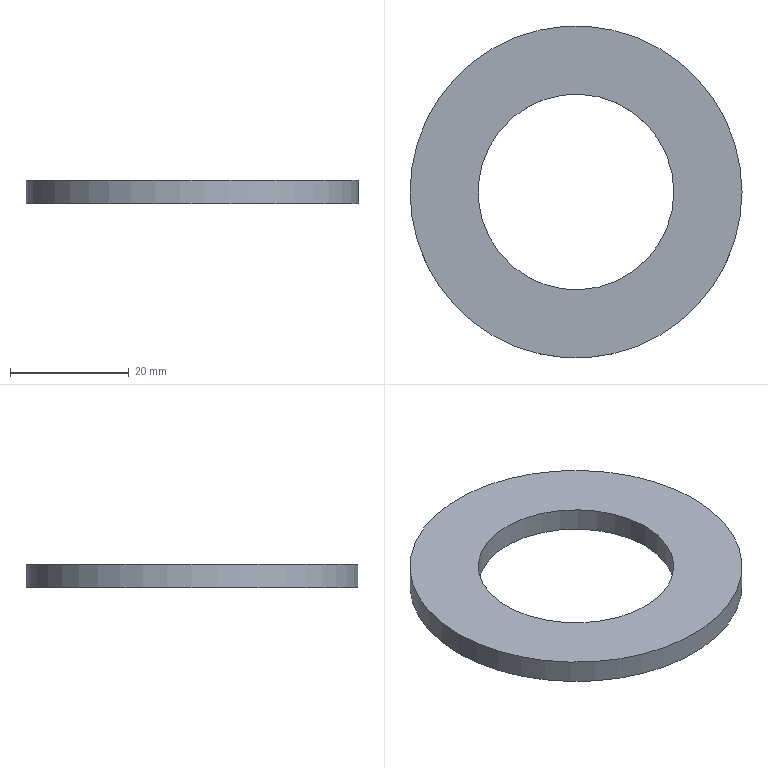Component | NX | GB-T95-2002_M30 | 1 solid | 4 faces | box 56 x 56 x 4 mm | volume 6431 mm3 | cylinder 2 | plane 2 | commonest cylinder face diameters 56 x1 33 x1
STEP:
#1=CARTESIAN_POINT('',(0.,0.,0.));
#2=DIRECTION('',(0.,0.,1.));
#3=DIRECTION('',(1.,0.,0.));
#4=AXIS2_PLACEMENT_3D('',#1,#2,#3);
#5=CARTESIAN_POINT('',(28.,0.,-9.));
#6=VERTEX_POINT('',#5);
#7=CARTESIAN_POINT('',(0.,0.,-9.));
#8=DIRECTION('',(0.,0.,1.));
#9=DIRECTION('',(1.,0.,0.));
#10=AXIS2_PLACEMENT_3D('',#7,#8,#9);
#11=CIRCLE('',#10,28.);
#12=CARTESIAN_POINT('',(0.,0.,-5.));
#13=DIRECTION('',(0.,0.,1.));
#14=DIRECTION('',(1.,0.,0.));
#15=AXIS2_PLACEMENT_3D('',#12,#13,#14);
#16=CYLINDRICAL_SURFACE('',#15,28.);
#17=CARTESIAN_POINT('',(0.,-4.));
#18=DIRECTION('',(1.,0.));
#19=VECTOR('',#18,1.);
#20=LINE('',#17,#19);
#21=(GEOMETRIC_REPRESENTATION_CONTEXT(2)PARAMETRIC_REPRESENTATION_CONTEXT()REPRESENTATION_CONTEXT('',''));
#22=DEFINITIONAL_REPRESENTATION('',(#20),#21);
#23=PCURVE('',#16,#22);
#24=CARTESIAN_POINT('',(-28.,0.,-9.));
#25=DIRECTION('',(0.,0.,-1.));
#26=DIRECTION('',(-1.,0.,0.));
#27=AXIS2_PLACEMENT_3D('',#24,#25,#26);
#28=PLANE('',#27);
#29=CARTESIAN_POINT('',(-56.,0.));
#30=CARTESIAN_POINT('',(-56.,48.497));
#31=CARTESIAN_POINT('',(-14.,24.249));
#32=CARTESIAN_POINT('',(28.,0.));
#33=CARTESIAN_POINT('',(-14.,-24.249));
#34=CARTESIAN_POINT('',(-56.,-48.497));
#35=CARTESIAN_POINT('',(-56.,0.));
#36=(BOUNDED_CURVE()B_SPLINE_CURVE(2,(#29,#30,#31,#32,#33,#34,#35),.UNSPECIFIED.,.T.,.F.)B_SPLINE_CURVE_WITH_KNOTS((1,2,2,2,2,1),(-2.094,0.,2.094,4.189,6.283,8.378),.UNSPECIFIED.)CURVE()GEOMETRIC_REPRESENTATION_ITEM()RATIONAL_B_SPLINE_CURVE((1.,0.5,1.,0.5,1.,0.5,1.))REPRESENTATION_ITEM(''));
#37=(GEOMETRIC_REPRESENTATION_CONTEXT(2)PARAMETRIC_REPRESENTATION_CONTEXT()REPRESENTATION_CONTEXT('',''));
#38=DEFINITIONAL_REPRESENTATION('',(#36),#37);
#39=PCURVE('',#28,#38);
#40=SURFACE_CURVE('',#11,(#23,#39),.PCURVE_S1.);
#41=EDGE_CURVE('',#6,#6,#40,.T.);
#42=ORIENTED_EDGE('',*,*,#41,.T.);
#43=CARTESIAN_POINT('',(28.,0.,-5.));
#44=VERTEX_POINT('',#43);
#45=CARTESIAN_POINT('',(28.,0.,-9.));
#46=CARTESIAN_POINT('',(28.,0.,-5.));
#47=B_SPLINE_CURVE_WITH_KNOTS('',1,(#45,#46),.UNSPECIFIED.,.F.,.F.,(2,2),(-4.,0.),.PIECEWISE_BEZIER_KNOTS.);
#48=CARTESIAN_POINT('',(6.283,0.));
#49=DIRECTION('',(0.,1.));
#50=VECTOR('',#49,1.);
#51=LINE('',#48,#50);
#52=(GEOMETRIC_REPRESENTATION_CONTEXT(2)PARAMETRIC_REPRESENTATION_CONTEXT()REPRESENTATION_CONTEXT('',''));
#53=DEFINITIONAL_REPRESENTATION('',(#51),#52);
#54=PCURVE('',#16,#53);
#55=CARTESIAN_POINT('',(0.,0.));
#56=DIRECTION('',(0.,1.));
#57=VECTOR('',#56,1.);
#58=LINE('',#55,#57);
#59=(GEOMETRIC_REPRESENTATION_CONTEXT(2)PARAMETRIC_REPRESENTATION_CONTEXT()REPRESENTATION_CONTEXT('',''));
#60=DEFINITIONAL_REPRESENTATION('',(#58),#59);
#61=PCURVE('',#16,#60);
#62=SEAM_CURVE('',#47,(#54,#61),.PCURVE_S1.);
#63=EDGE_CURVE('',#6,#44,#62,.T.);
#64=ORIENTED_EDGE('',*,*,#63,.T.);
#65=CARTESIAN_POINT('',(0.,0.,-5.));
#66=DIRECTION('',(0.,0.,1.));
#67=DIRECTION('',(1.,0.,0.));
#68=AXIS2_PLACEMENT_3D('',#65,#66,#67);
#69=CIRCLE('',#68,28.);
#70=CARTESIAN_POINT('',(0.,0.));
#71=DIRECTION('',(1.,0.));
#72=VECTOR('',#71,1.);
#73=LINE('',#70,#72);
#74=(GEOMETRIC_REPRESENTATION_CONTEXT(2)PARAMETRIC_REPRESENTATION_CONTEXT()REPRESENTATION_CONTEXT('',''));
#75=DEFINITIONAL_REPRESENTATION('',(#73),#74);
#76=PCURVE('',#16,#75);
#77=CARTESIAN_POINT('',(-16.5,0.,-5.));
#78=DIRECTION('',(0.,0.,1.));
#79=DIRECTION('',(1.,0.,0.));
#80=AXIS2_PLACEMENT_3D('',#77,#78,#79);
#81=PLANE('',#80);
#82=CARTESIAN_POINT('',(16.5,0.));
#83=DIRECTION('',(1.,0.));
#84=AXIS2_PLACEMENT_2D('',#82,#83);
#85=CIRCLE('',#84,28.);
#86=(GEOMETRIC_REPRESENTATION_CONTEXT(2)PARAMETRIC_REPRESENTATION_CONTEXT()REPRESENTATION_CONTEXT('',''));
#87=DEFINITIONAL_REPRESENTATION('',(#85),#86);
#88=PCURVE('',#81,#87);
#89=SURFACE_CURVE('',#69,(#76,#88),.PCURVE_S1.);
#90=EDGE_CURVE('',#44,#44,#89,.T.);
#91=ORIENTED_EDGE('',*,*,#90,.F.);
#92=ORIENTED_EDGE('',*,*,#63,.F.);
#93=EDGE_LOOP('',(#42,#64,#91,#92));
#94=FACE_BOUND('',#93,.T.);
#95=ADVANCED_FACE('',(#94),#16,.T.);
#96=CARTESIAN_POINT('',(16.5,0.,-9.));
#97=VERTEX_POINT('',#96);
#98=CARTESIAN_POINT('',(0.,0.,-9.));
#99=DIRECTION('',(0.,0.,1.));
#100=DIRECTION('',(1.,0.,0.));
#101=AXIS2_PLACEMENT_3D('',#98,#99,#100);
#102=CIRCLE('',#101,16.5);
#103=CARTESIAN_POINT('',(-44.5,0.));
#104=CARTESIAN_POINT('',(-44.5,28.579));
#105=CARTESIAN_POINT('',(-19.75,14.289));
#106=CARTESIAN_POINT('',(5.,0.));
#107=CARTESIAN_POINT('',(-19.75,-14.289));
#108=CARTESIAN_POINT('',(-44.5,-28.579));
#109=CARTESIAN_POINT('',(-44.5,0.));
#110=(BOUNDED_CURVE()B_SPLINE_CURVE(2,(#103,#104,#105,#106,#107,#108,#109),.UNSPECIFIED.,.T.,.F.)B_SPLINE_CURVE_WITH_KNOTS((1,2,2,2,2,1),(-2.094,0.,2.094,4.189,6.283,8.378),.UNSPECIFIED.)CURVE()GEOMETRIC_REPRESENTATION_ITEM()RATIONAL_B_SPLINE_CURVE((1.,0.5,1.,0.5,1.,0.5,1.))REPRESENTATION_ITEM(''));
#111=(GEOMETRIC_REPRESENTATION_CONTEXT(2)PARAMETRIC_REPRESENTATION_CONTEXT()REPRESENTATION_CONTEXT('',''));
#112=DEFINITIONAL_REPRESENTATION('',(#110),#111);
#113=PCURVE('',#28,#112);
#114=CARTESIAN_POINT('',(0.,0.,-5.));
#115=DIRECTION('',(0.,0.,1.));
#116=DIRECTION('',(1.,0.,0.));
#117=AXIS2_PLACEMENT_3D('',#114,#115,#116);
#118=CYLINDRICAL_SURFACE('',#117,16.5);
#119=CARTESIAN_POINT('',(0.,-4.));
#120=DIRECTION('',(1.,0.));
#121=VECTOR('',#120,1.);
#122=LINE('',#119,#121);
#123=(GEOMETRIC_REPRESENTATION_CONTEXT(2)PARAMETRIC_REPRESENTATION_CONTEXT()REPRESENTATION_CONTEXT('',''));
#124=DEFINITIONAL_REPRESENTATION('',(#122),#123);
#125=PCURVE('',#118,#124);
#126=SURFACE_CURVE('',#102,(#113,#125),.PCURVE_S1.);
#127=EDGE_CURVE('',#97,#97,#126,.T.);
#128=ORIENTED_EDGE('',*,*,#127,.T.);
#129=EDGE_LOOP('',(#128));
#130=FACE_BOUND('',#129,.T.);
#131=ORIENTED_EDGE('',*,*,#41,.F.);
#132=EDGE_LOOP('',(#131));
#133=FACE_BOUND('',#132,.T.);
#134=ADVANCED_FACE('',(#130,#133),#28,.T.);
#135=CARTESIAN_POINT('',(16.5,0.,-5.));
#136=VERTEX_POINT('',#135);
#137=CARTESIAN_POINT('',(0.,0.,-5.));
#138=DIRECTION('',(0.,0.,1.));
#139=DIRECTION('',(1.,0.,0.));
#140=AXIS2_PLACEMENT_3D('',#137,#138,#139);
#141=CIRCLE('',#140,16.5);
#142=CARTESIAN_POINT('',(0.,0.));
#143=DIRECTION('',(1.,0.));
#144=VECTOR('',#143,1.);
#145=LINE('',#142,#144);
#146=(GEOMETRIC_REPRESENTATION_CONTEXT(2)PARAMETRIC_REPRESENTATION_CONTEXT()REPRESENTATION_CONTEXT('',''));
#147=DEFINITIONAL_REPRESENTATION('',(#145),#146);
#148=PCURVE('',#118,#147);
#149=CARTESIAN_POINT('',(16.5,0.));
#150=DIRECTION('',(1.,0.));
#151=AXIS2_PLACEMENT_2D('',#149,#150);
#152=CIRCLE('',#151,16.5);
#153=(GEOMETRIC_REPRESENTATION_CONTEXT(2)PARAMETRIC_REPRESENTATION_CONTEXT()REPRESENTATION_CONTEXT('',''));
#154=DEFINITIONAL_REPRESENTATION('',(#152),#153);
#155=PCURVE('',#81,#154);
#156=SURFACE_CURVE('',#141,(#148,#155),.PCURVE_S1.);
#157=EDGE_CURVE('',#136,#136,#156,.T.);
#158=ORIENTED_EDGE('',*,*,#157,.F.);
#159=CARTESIAN_POINT('',(16.5,-0.,-9.));
#160=CARTESIAN_POINT('',(16.5,-0.,-5.));
#161=B_SPLINE_CURVE_WITH_KNOTS('',1,(#159,#160),.UNSPECIFIED.,.F.,.F.,(2,2),(-4.,0.),.PIECEWISE_BEZIER_KNOTS.);
#162=CARTESIAN_POINT('',(0.,0.));
#163=DIRECTION('',(0.,1.));
#164=VECTOR('',#163,1.);
#165=LINE('',#162,#164);
#166=(GEOMETRIC_REPRESENTATION_CONTEXT(2)PARAMETRIC_REPRESENTATION_CONTEXT()REPRESENTATION_CONTEXT('',''));
#167=DEFINITIONAL_REPRESENTATION('',(#165),#166);
#168=PCURVE('',#118,#167);
#169=CARTESIAN_POINT('',(6.283,0.));
#170=DIRECTION('',(0.,1.));
#171=VECTOR('',#170,1.);
#172=LINE('',#169,#171);
#173=(GEOMETRIC_REPRESENTATION_CONTEXT(2)PARAMETRIC_REPRESENTATION_CONTEXT()REPRESENTATION_CONTEXT('',''));
#174=DEFINITIONAL_REPRESENTATION('',(#172),#173);
#175=PCURVE('',#118,#174);
#176=SEAM_CURVE('',#161,(#168,#175),.PCURVE_S1.);
#177=EDGE_CURVE('',#97,#136,#176,.T.);
#178=ORIENTED_EDGE('',*,*,#177,.F.);
#179=ORIENTED_EDGE('',*,*,#127,.T.);
#180=ORIENTED_EDGE('',*,*,#177,.T.);
#181=EDGE_LOOP('',(#158,#178,#179,#180));
#182=FACE_BOUND('',#181,.F.);
#183=ADVANCED_FACE('',(#182),#118,.F.);
#184=ORIENTED_EDGE('',*,*,#90,.T.);
#185=EDGE_LOOP('',(#184));
#186=FACE_BOUND('',#185,.T.);
#187=ORIENTED_EDGE('',*,*,#157,.F.);
#188=EDGE_LOOP('',(#187));
#189=FACE_BOUND('',#188,.T.);
#190=ADVANCED_FACE('',(#186,#189),#81,.T.);
#191=CLOSED_SHELL('',(#95,#134,#183,#190));
#192=MANIFOLD_SOLID_BREP('',#191);
#193=(LENGTH_UNIT()NAMED_UNIT(*)SI_UNIT(.MILLI.,.METRE.));
#194=UNCERTAINTY_MEASURE_WITH_UNIT(LENGTH_MEASURE(0.00001),#193,'','');
#195=(NAMED_UNIT(*)PLANE_ANGLE_UNIT()SI_UNIT($,.RADIAN.));
#196=(NAMED_UNIT(*)SI_UNIT($,.STERADIAN.)SOLID_ANGLE_UNIT());
#197=(GEOMETRIC_REPRESENTATION_CONTEXT(3)GLOBAL_UNCERTAINTY_ASSIGNED_CONTEXT((#194))GLOBAL_UNIT_ASSIGNED_CONTEXT((#193,#195,#196))REPRESENTATION_CONTEXT('',''));
#198=ADVANCED_BREP_SHAPE_REPRESENTATION('',(#4,#192),#197);